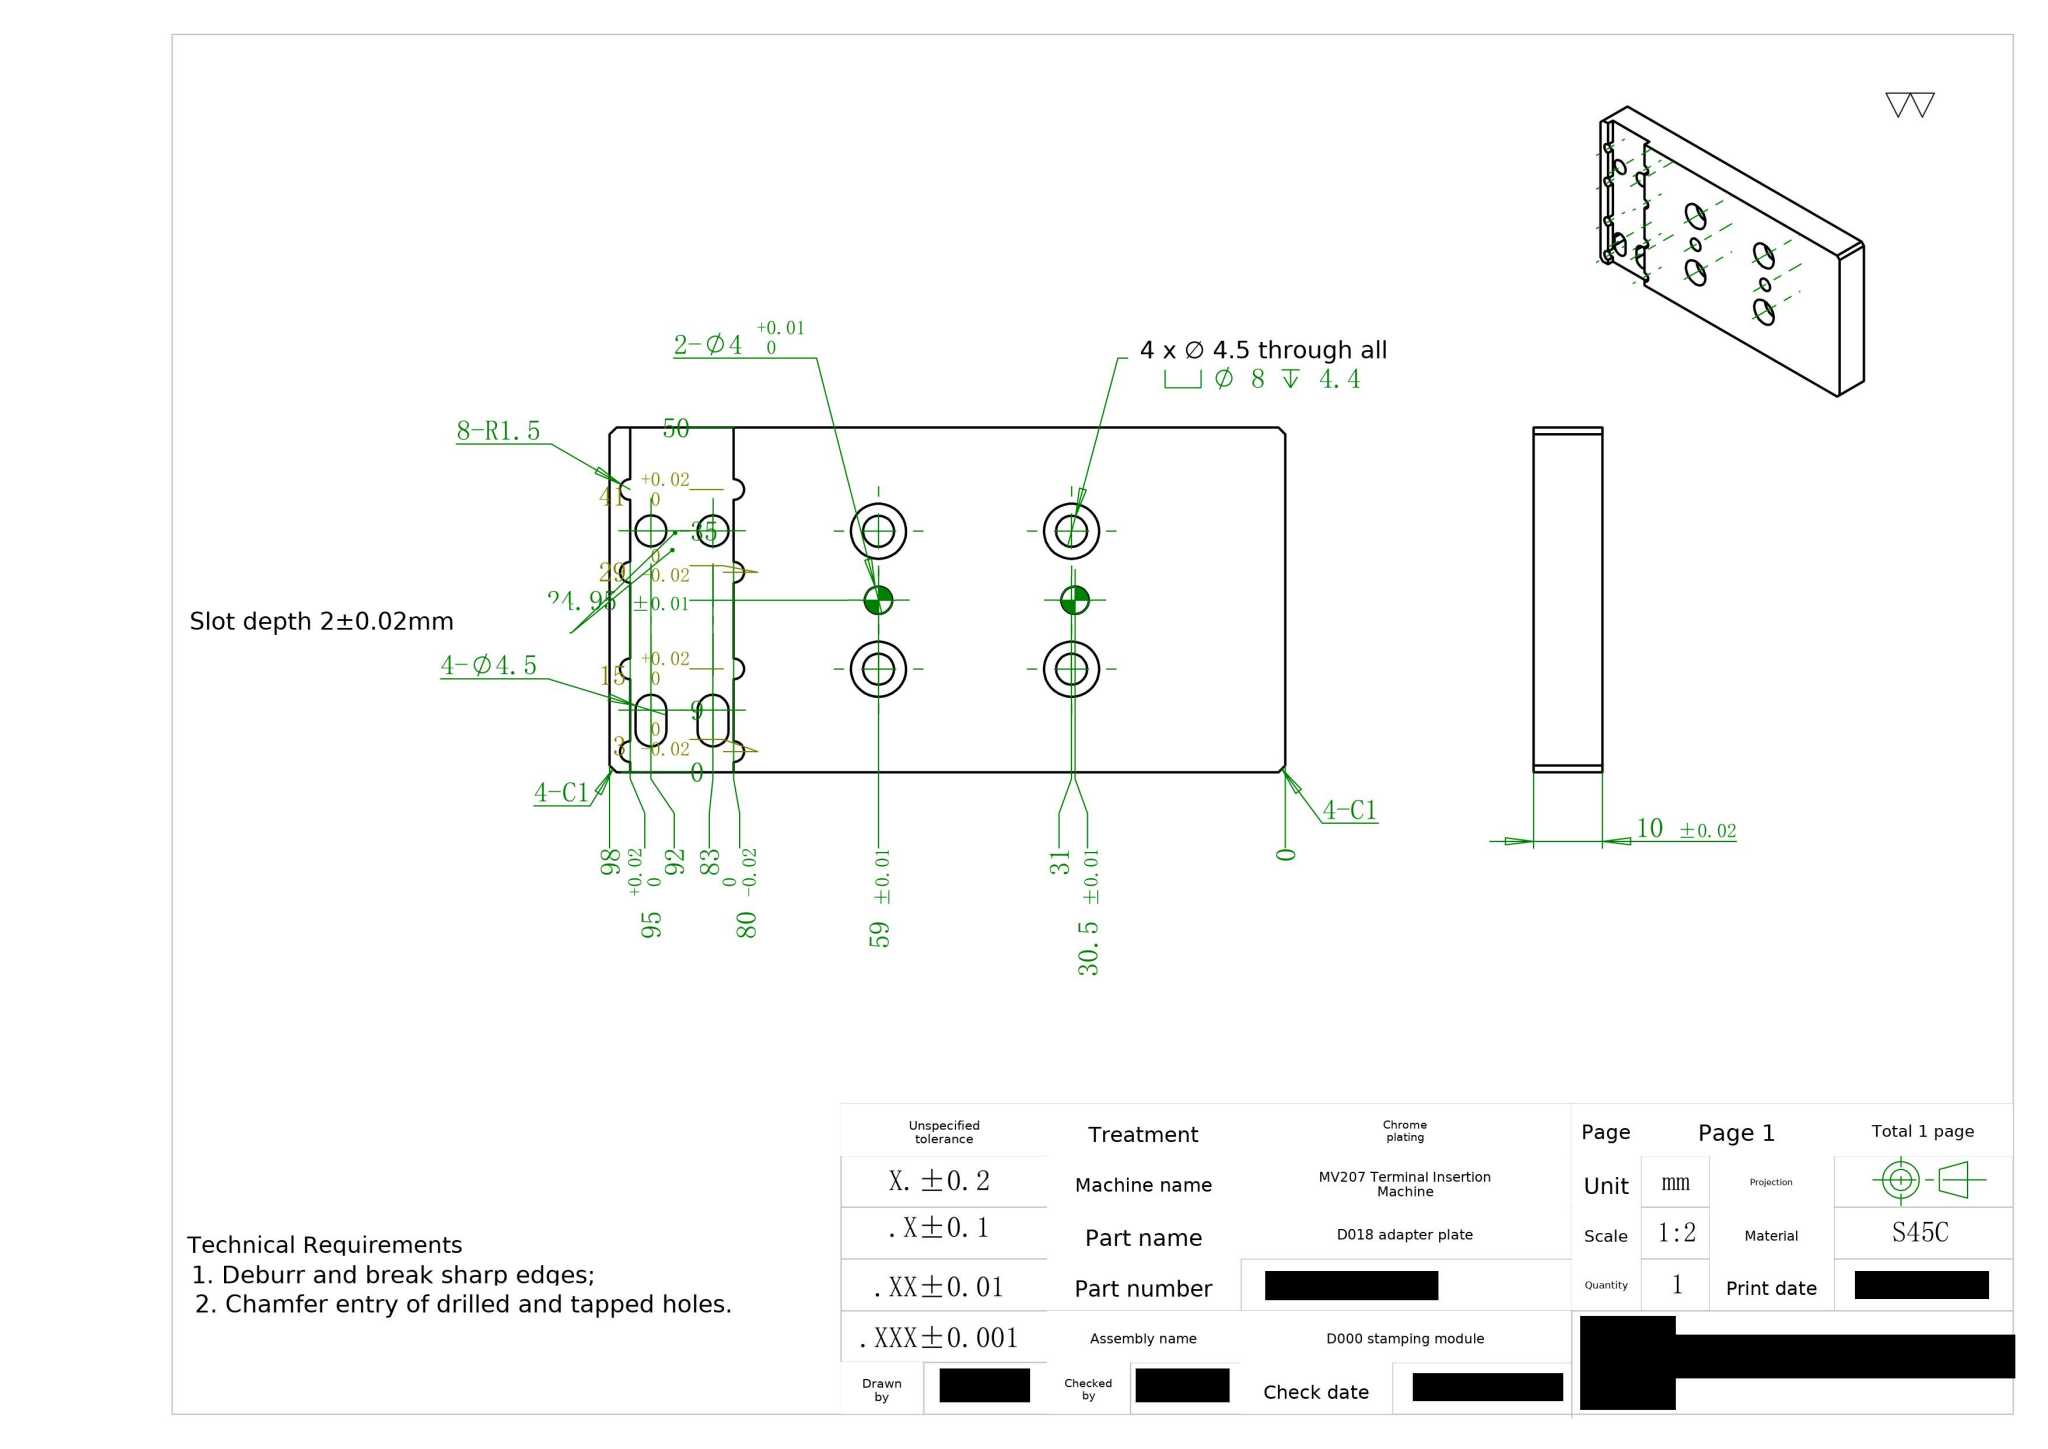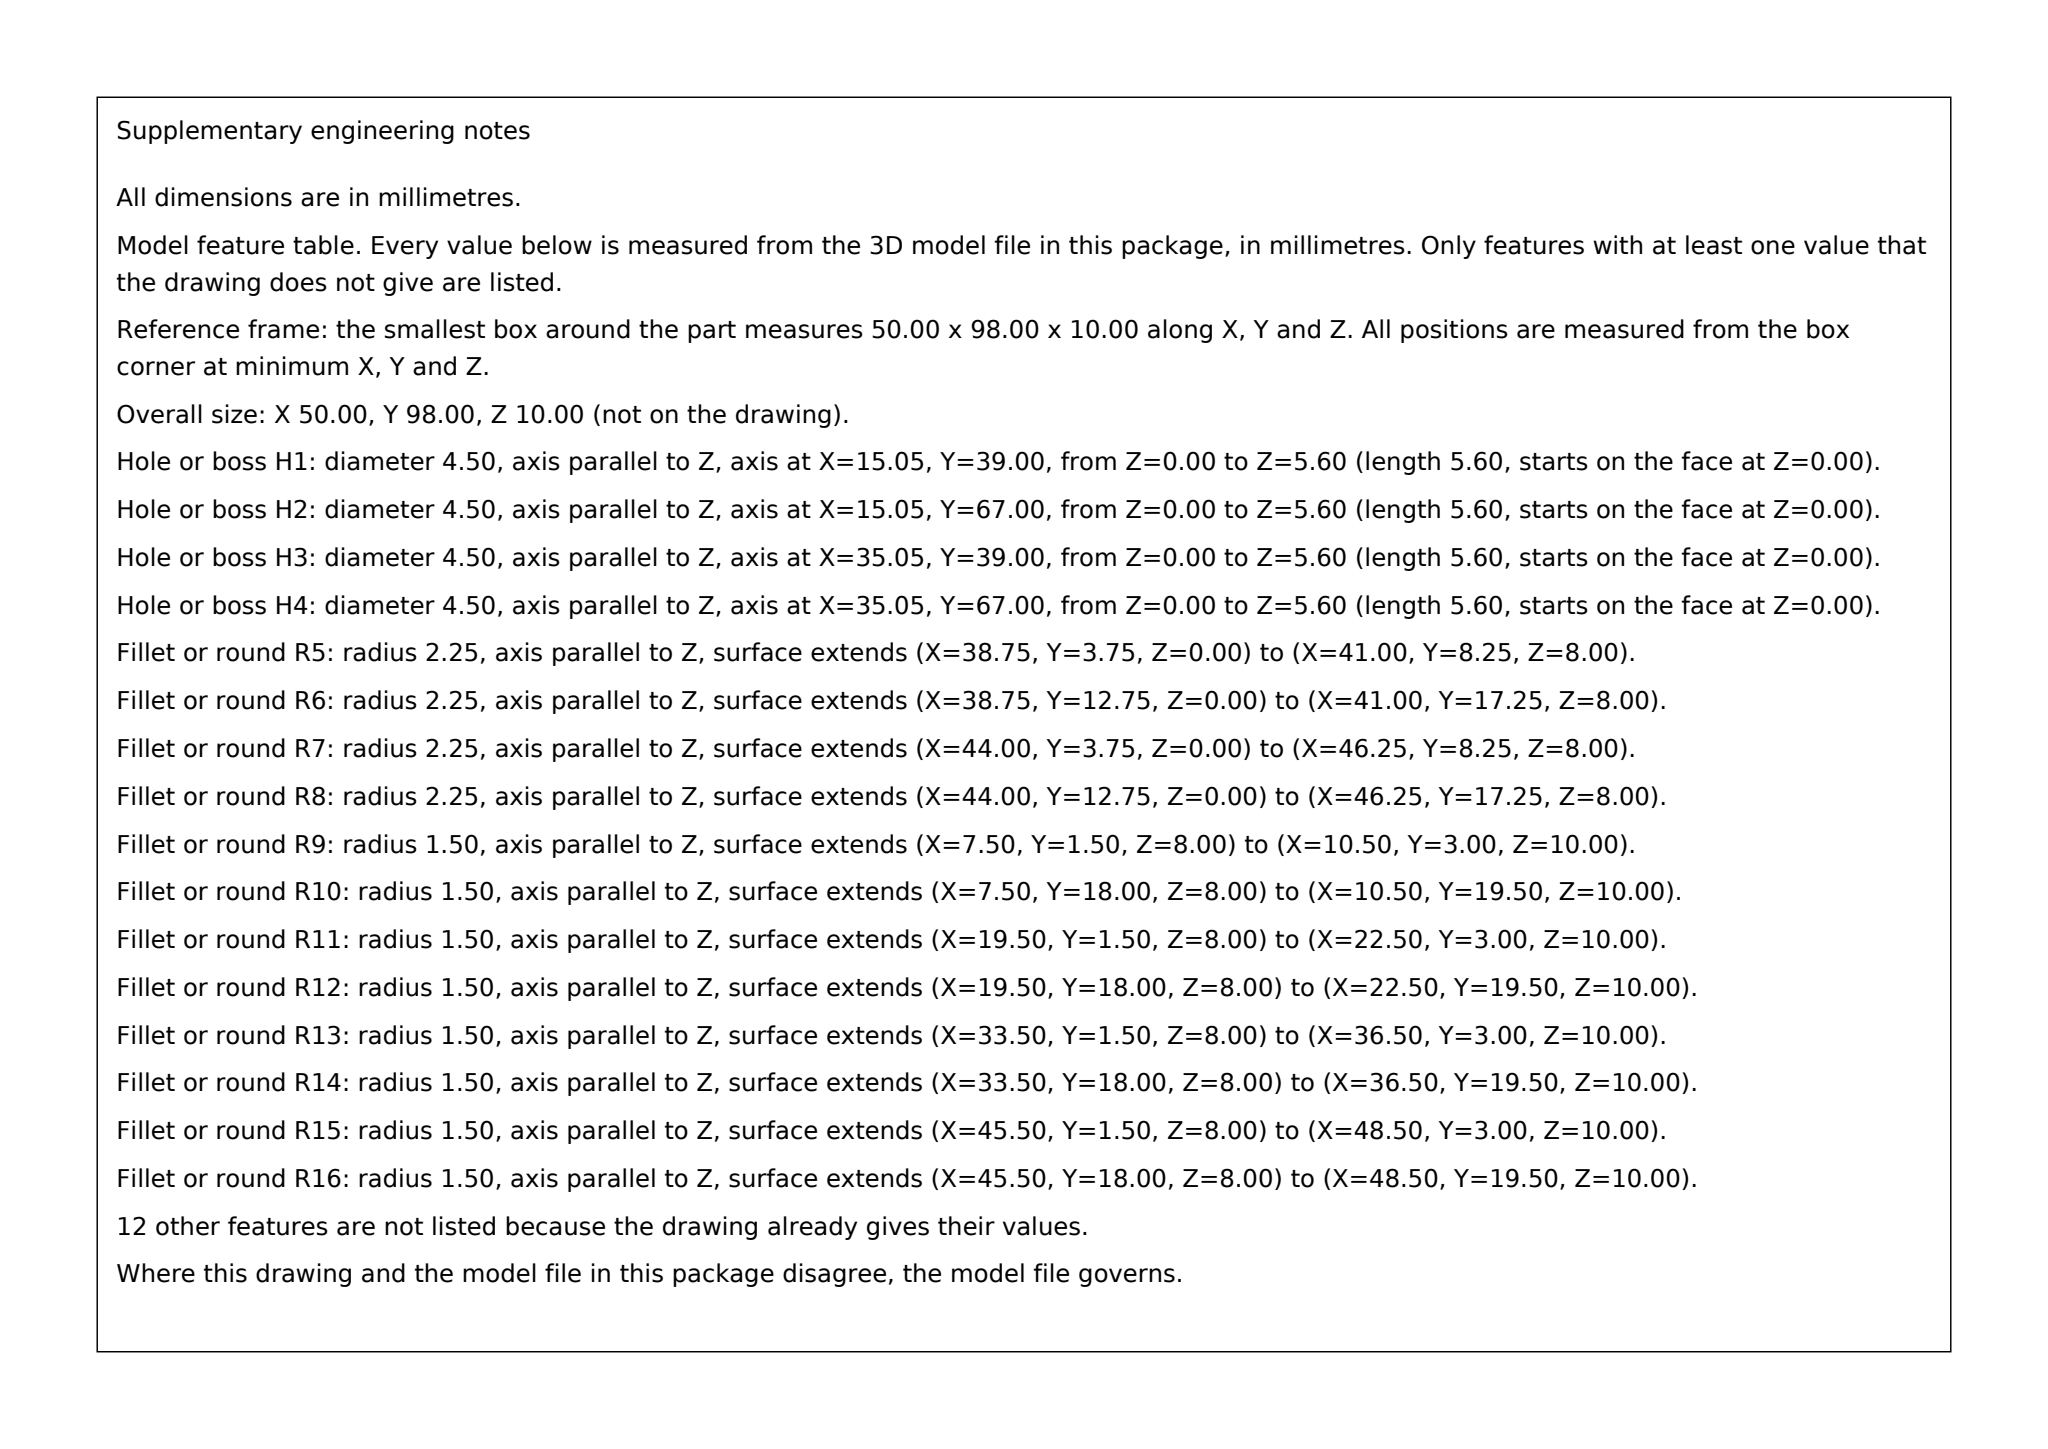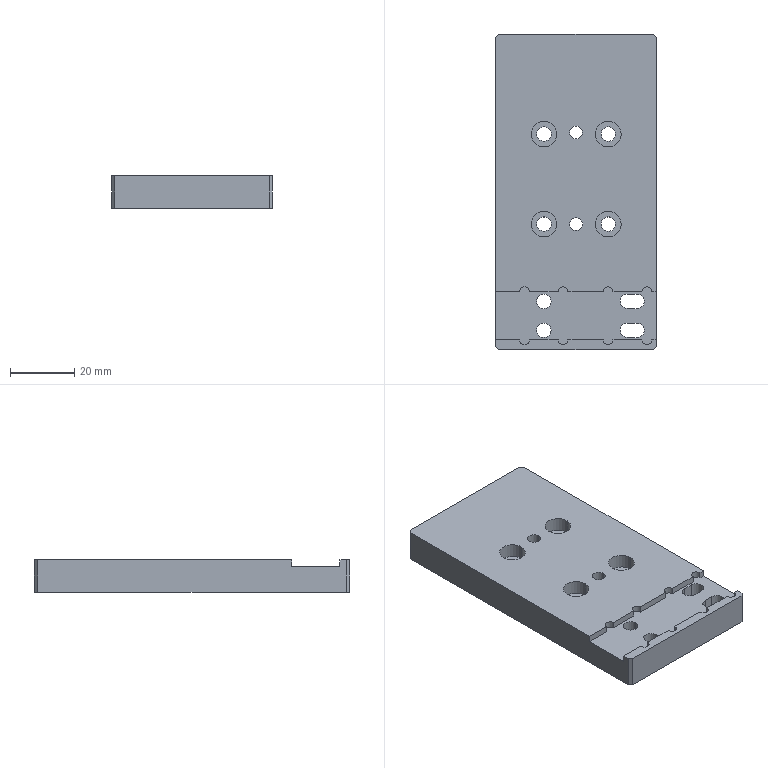Part | SolidWorks | mm | material S45C | 1 solid | 68 faces | box 50 x 98 x 10 mm | volume 45206 mm3 | cylinder 38 | plane 30 | commonest cylinder face diameters 4.5 x18 8 x8 3 x8 4 x4
build123d program:
from build123d import *

# Parameters (mm, degrees)
SKETCH1_W                                       = 50
SKETCH1_H                                       = 98
BOSS_EXTRUDE1_DEPTH                             = 10
SKETCH3_W                                       = 12
SKETCH3_H                                       = 15
CUT_EXTRUDE2_DEPTH                              = 2
SKETCH4_R                                       = 1.5
CUT_EXTRUDE3_DEPTH                              = 2
F_4_5_4_5_DIAMETER_HOLE1_D                      = 4.5
M4_HEX_SOCKET_HEAD_CAP_SCREW_CBORE2_D           = 4.5
M4_HEX_SOCKET_HEAD_CAP_SCREW_CBORE2_CBORE_D     = 8
M4_HEX_SOCKET_HEAD_CAP_SCREW_CBORE2_CBORE_DEPTH = 4.4
F_4_0_4_DIAMETER_HOLE1_D                        = 4
LPATTERN1_COUNT                                 = 2
LPATTERN1_PITCH                                 = 26
CHAMFER1_SIZE                                   = 1
CUT_EXTRUDE4_START                              = -2
SKETCH12_W                                      = 50
SKETCH12_H                                      = 15
CUT_EXTRUDE4_DEPTH                              = 2
CUT_EXTRUDE5_DEPTH                              = 56.911


with BuildPart() as part:
    # Sketch1 → Boss-Extrude1 (new body)
    with BuildSketch(Plane.XY):
        Rectangle(SKETCH1_W, SKETCH1_H)
    extrude(amount=BOSS_EXTRUDE1_DEPTH)

    # Sketch3 → Cut-Extrude2 (cut)
    with BuildSketch(Plane.XY.offset(10)):
        with Locations((16, -38.5)):
            Rectangle(SKETCH3_W, SKETCH3_H)
    cut_extrude2 = extrude(amount=-CUT_EXTRUDE2_DEPTH, mode=Mode.SUBTRACT)

    # Sketch4 → Cut-Extrude3 (cut)
    with BuildSketch(Plane.XY.offset(10)):
        with Locations((10, -46)):
            Circle(SKETCH4_R)
        with Locations((10, -31)):
            Circle(SKETCH4_R)
        with Locations((22, -31)):
            Circle(SKETCH4_R)
        with Locations((22, -46)):
            Circle(SKETCH4_R)
    cut_extrude3 = extrude(amount=-CUT_EXTRUDE3_DEPTH, mode=Mode.SUBTRACT)

    # 4.5 _4.5_ Diameter Hole1 (through all)
    with Locations(Plane(origin=(0, 0, 0), x_dir=(-1, 0, 0), z_dir=(0, 0, -1))):
        with Locations((-16, -34), (-16, -43)):
            f_4_5_4_5_diameter_hole1 = Hole(F_4_5_4_5_DIAMETER_HOLE1_D / 2)

    # M4 Hex Socket Head Cap Screw CBORE2 (through all)
    with Locations(Plane.XY.offset(10)):
        with Locations((-9.95, -10), (-9.95, 18), (10.05, 18), (10.05, -10)):
            CounterBoreHole(M4_HEX_SOCKET_HEAD_CAP_SCREW_CBORE2_D / 2, M4_HEX_SOCKET_HEAD_CAP_SCREW_CBORE2_CBORE_D / 2, M4_HEX_SOCKET_HEAD_CAP_SCREW_CBORE2_CBORE_DEPTH)

    # 4.0 _4_ Diameter Hole1 (through all)
    with Locations(Plane.XY.offset(10)):
        with Locations((0.05, -10), (0.05, 18.5)):
            Hole(F_4_0_4_DIAMETER_HOLE1_D / 2)

    # LPattern1: Cut-Extrude2, Cut-Extrude3, 4.5 _4.5_ Diameter Hole1 ×2
    with Locations(*[(-i * LPATTERN1_PITCH, 0, 0) for i in range(1, LPATTERN1_COUNT)]):
        add(cut_extrude2, mode=Mode.SUBTRACT)
        add(cut_extrude3, mode=Mode.SUBTRACT)
        add(f_4_5_4_5_diameter_hole1, mode=Mode.SUBTRACT)

    # Chamfer1
    chamfer1_edges = [part.edges().sort_by_distance(p)[0] for p in [
        (25, -49, 5),
        (-25, -49, 5),
        (-25, 49, 5),
        (25, 49, 5),
    ]]
    chamfer(chamfer1_edges, length=CHAMFER1_SIZE)

    # Sketch12 → Cut-Extrude4 (cut)
    with BuildSketch(Plane.XY.offset(10).offset(CUT_EXTRUDE4_START)):
        with Locations((0, -38.5)):
            Rectangle(SKETCH12_W, SKETCH12_H)
    extrude(amount=CUT_EXTRUDE4_DEPTH, mode=Mode.SUBTRACT)

    # Sketch13 → Cut-Extrude5 (cut, through all)
    with BuildSketch(Plane(origin=(0, 0, 0), x_dir=(-1, 0, 0), z_dir=(0, 0, -1))):
        with BuildLine():
            Line((-16, -45.25), (-19, -45.25))
            ThreePointArc((-19, -45.25), (-21.25, -43), (-19, -40.75))
            Line((-19, -40.75), (-16, -40.75))
            ThreePointArc((-16, -40.75), (-13.75, -43), (-16, -45.25))
        make_face()
        with BuildLine():
            Line((-16, -36.25), (-19, -36.25))
            ThreePointArc((-19, -36.25), (-21.25, -34), (-19, -31.75))
            Line((-19, -31.75), (-16, -31.75))
            ThreePointArc((-16, -31.75), (-13.75, -34), (-16, -36.25))
        make_face()
    extrude(amount=-CUT_EXTRUDE5_DEPTH, mode=Mode.SUBTRACT)


solid = part.part